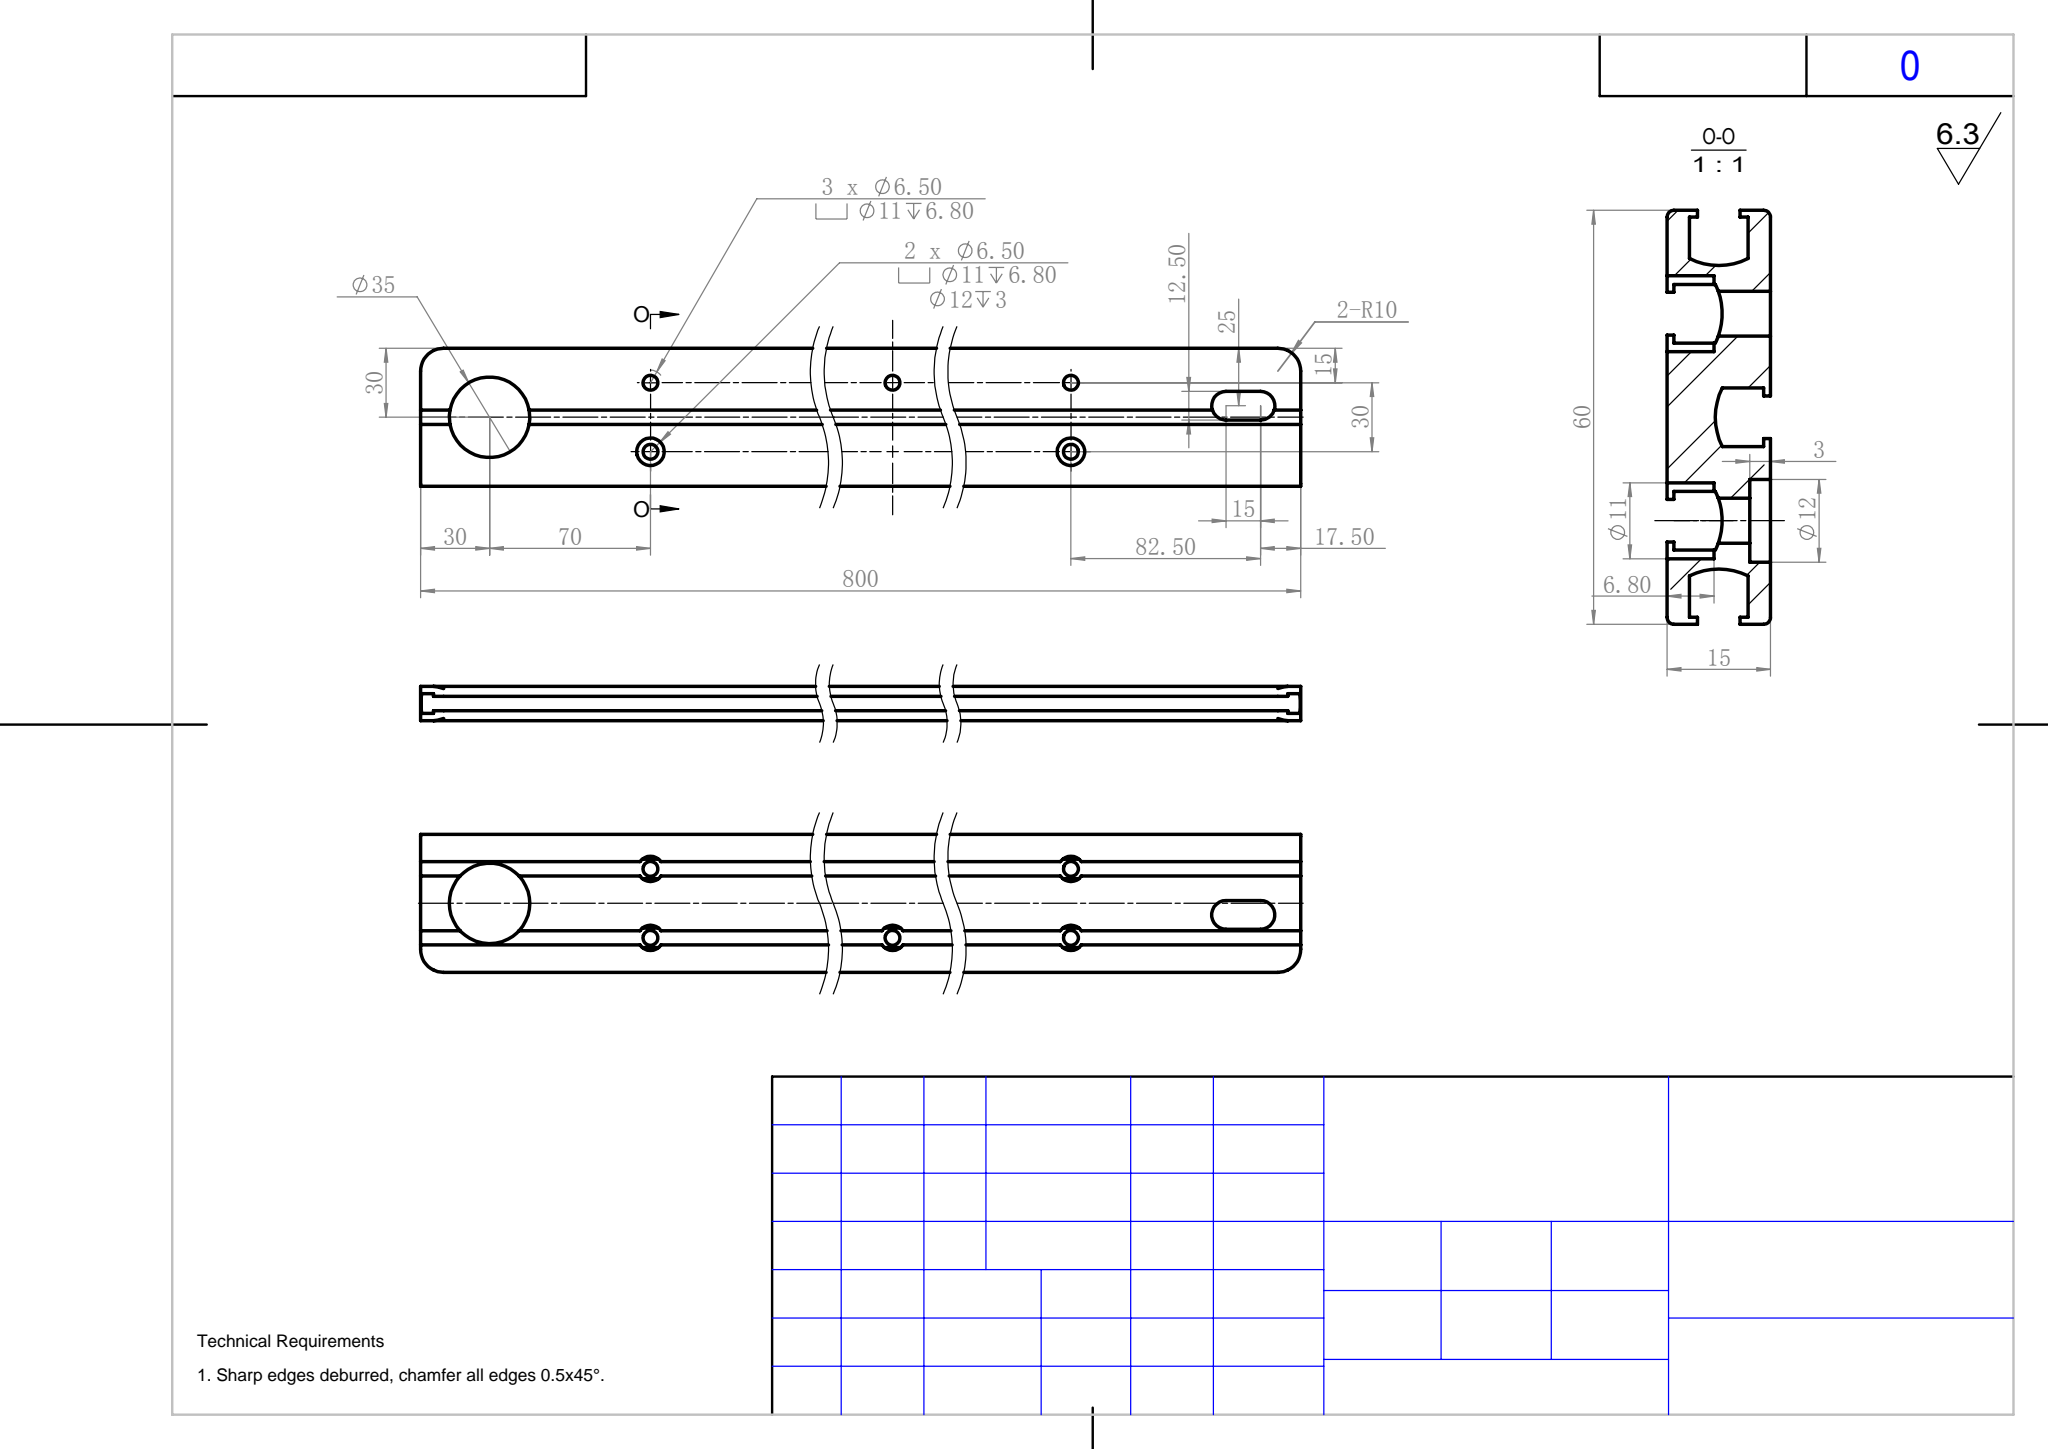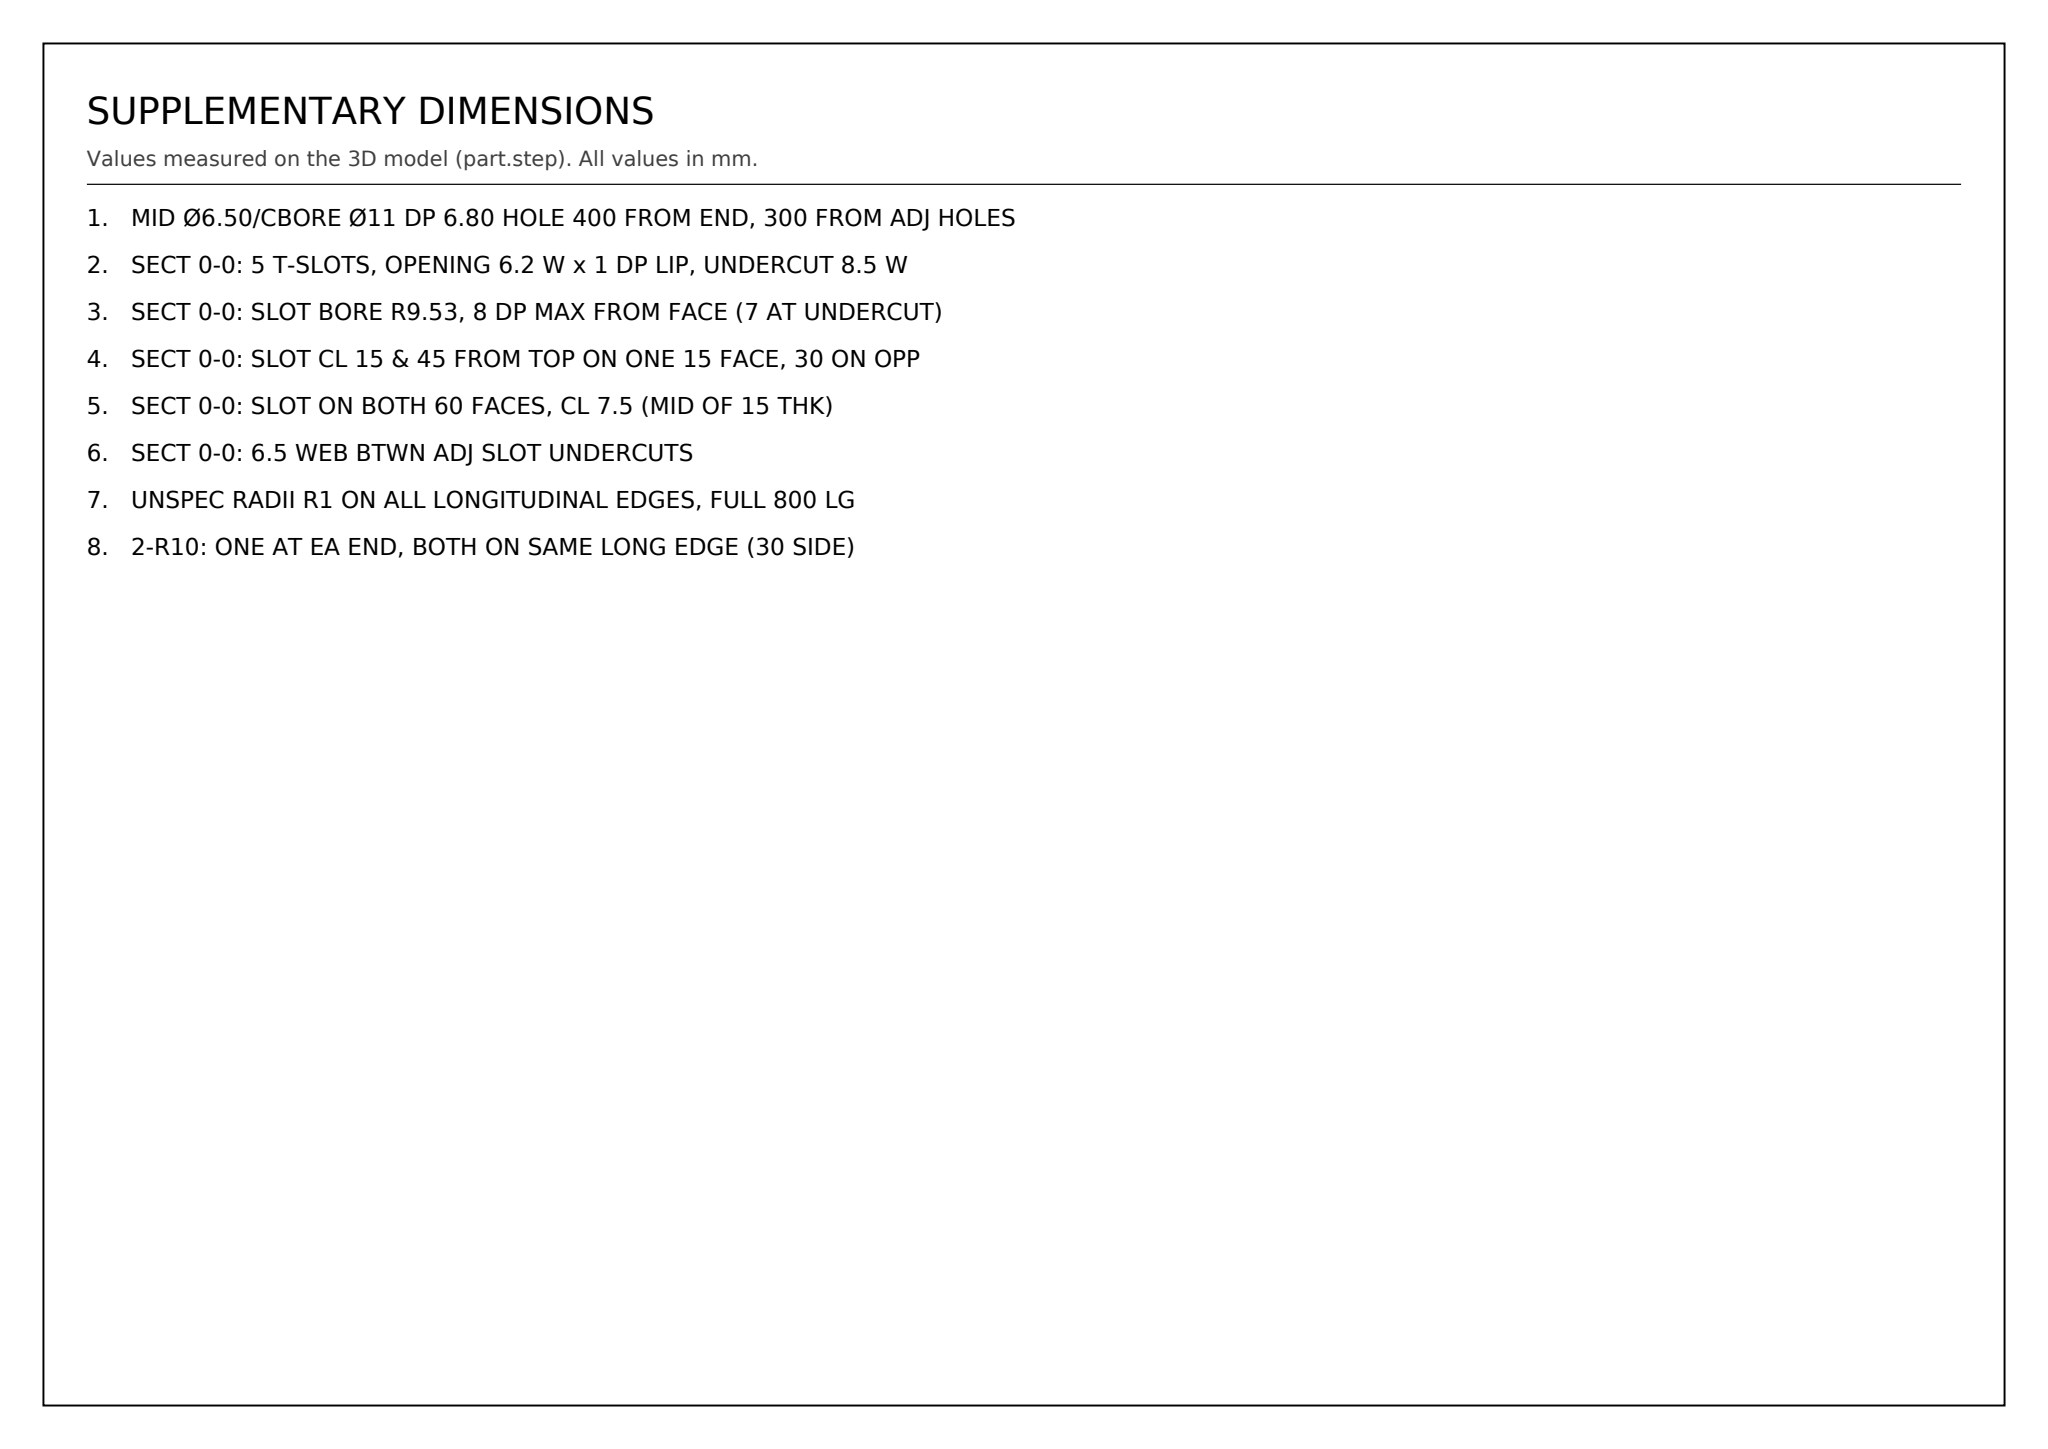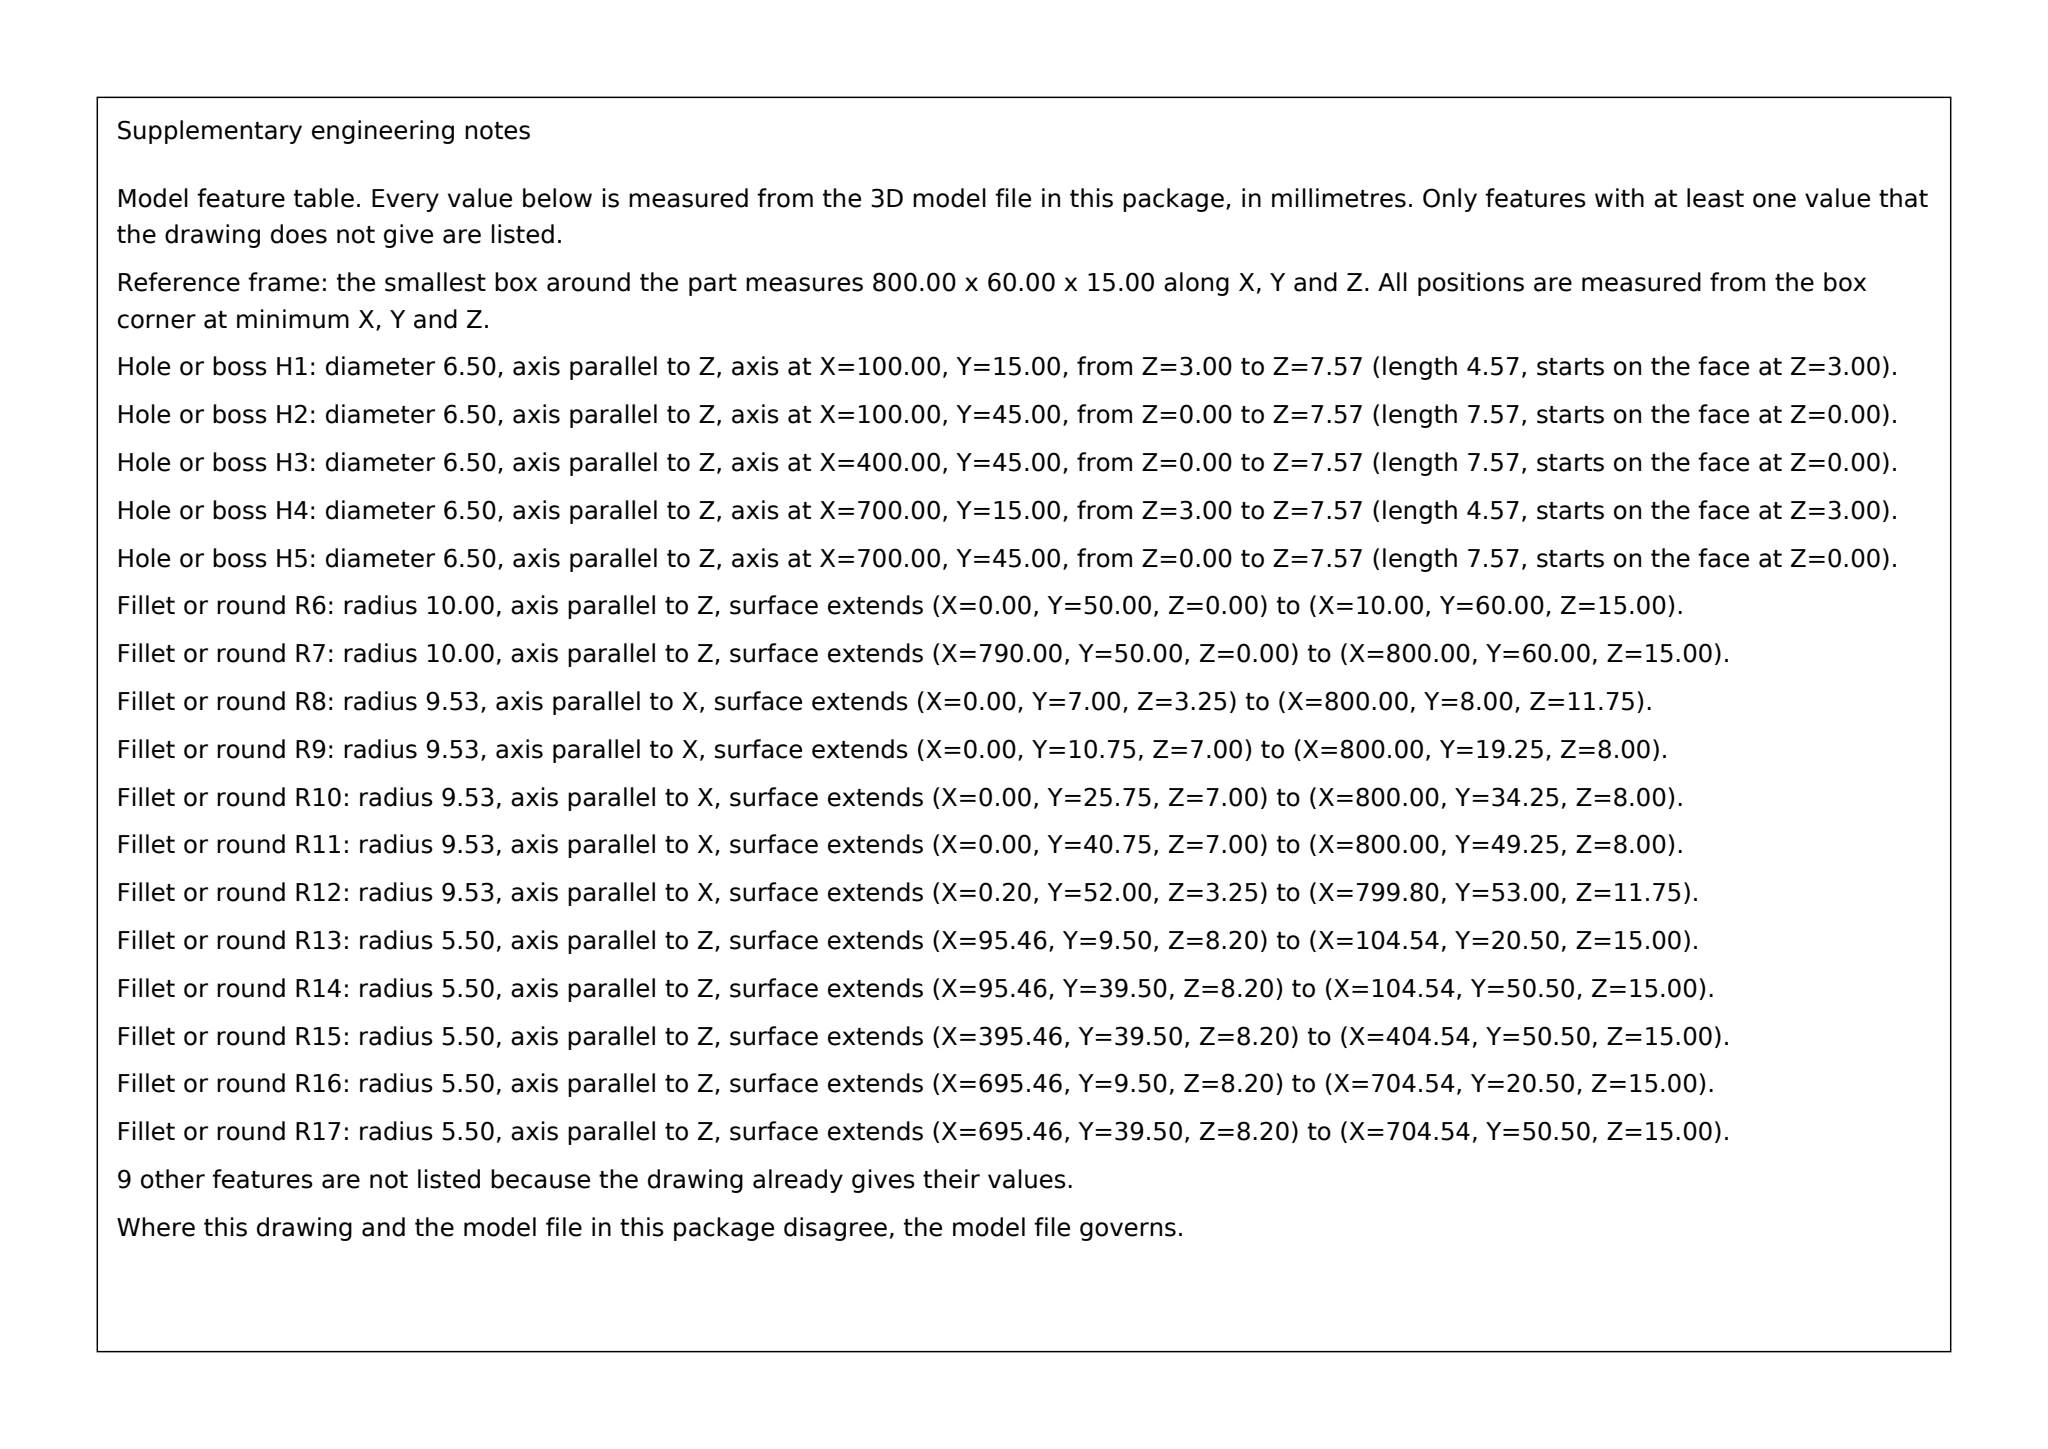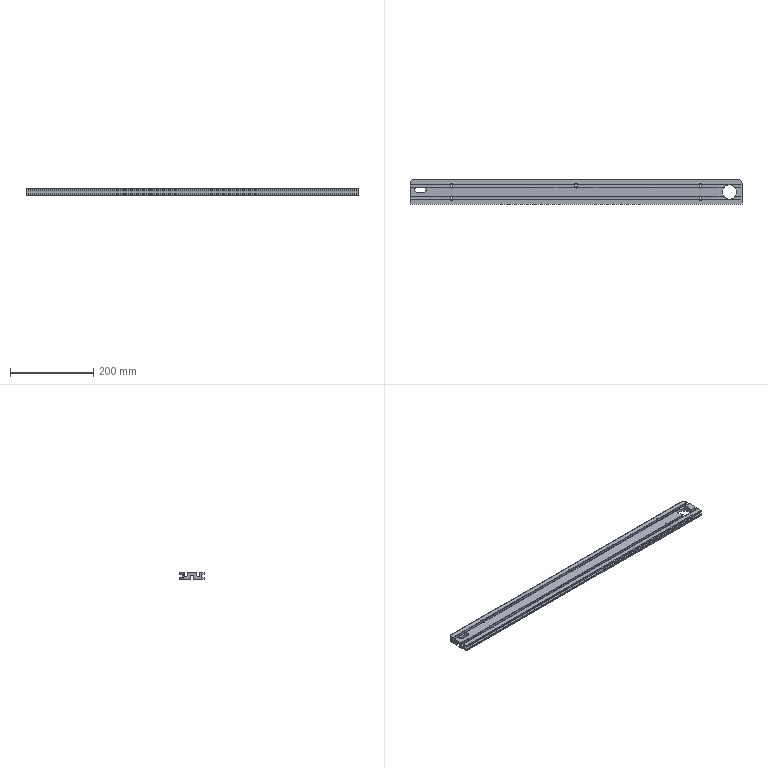Part | SolidWorks | mm | 1 solid | 142 faces | box 800 x 60 x 15 mm | volume 451229 mm3 | plane 93 | cylinder 49 | commonest cylinder face diameters 11 x15 6.5 x10 19.062 x7 12 x4 2 x4 12.5 x3 35 x2 19.063 x2
Drawing notes:
MID Ø6.50/CBORE Ø11 DP 6.80 HOLE 400 FROM END, 300 FROM ADJ HOLES | from the solid: Ø6.5+Ø11 c'bores on y=45 row at x=100, 400, 700; 400 is midway
SECT 0-0: 5 T-SLOTS, OPENING 6.2 W x 1 DP LIP, UNDERCUT 8.5 W | from the solid: y planes 11.9/18.1, 26.9/33.1, 41.9/48.1 =6.2; 10.75/19.25, 25.75/34.25, 40.75/49.25 =8.5; lip planes y=1.0, y=59.0, z=1.0, z=14.0
SECT 0-0: SLOT BORE R9.53, 8 DP MAX FROM FACE (7 AT UNDERCUT) | from the solid: x-axis cyl Ø19.062 at y=-1.53/61.53 (z=7.5) and z=-1.53/16.53: 9.531-1.53=8.0 deep, 7.0 at 4.25 offset
SECT 0-0: SLOT CL 15 & 45 FROM TOP ON ONE 15 FACE, 30 ON OPP | from the solid: Ø19.063 slot bores at (y=15,z=16.53) & (y=45,z=16.53); (y=30,z=-1.53)
SECT 0-0: SLOT ON BOTH 60 FACES, CL 7.5 (MID OF 15 THK) | from the solid: Ø19.062 slot bores at (y=-1.53,z=7.5) and (y=61.53,z=7.5)
SECT 0-0: 6.5 WEB BTWN ADJ SLOT UNDERCUTS | from the solid: undercut walls y=19.25/25.75 and y=34.25/40.75 => 6.5
UNSPEC RADII R1 ON ALL LONGITUDINAL EDGES, FULL 800 LG | from the solid: x-axis Ø2.0 cyls at (y1,z1),(y1,z14),(y59,z1),(y59,z14), L=800
2-R10: ONE AT EA END, BOTH ON SAME LONG EDGE (30 SIDE) | from the solid: z-axis Ø20 cyls at (x=10,y=50) and (x=790,y=50), L=15